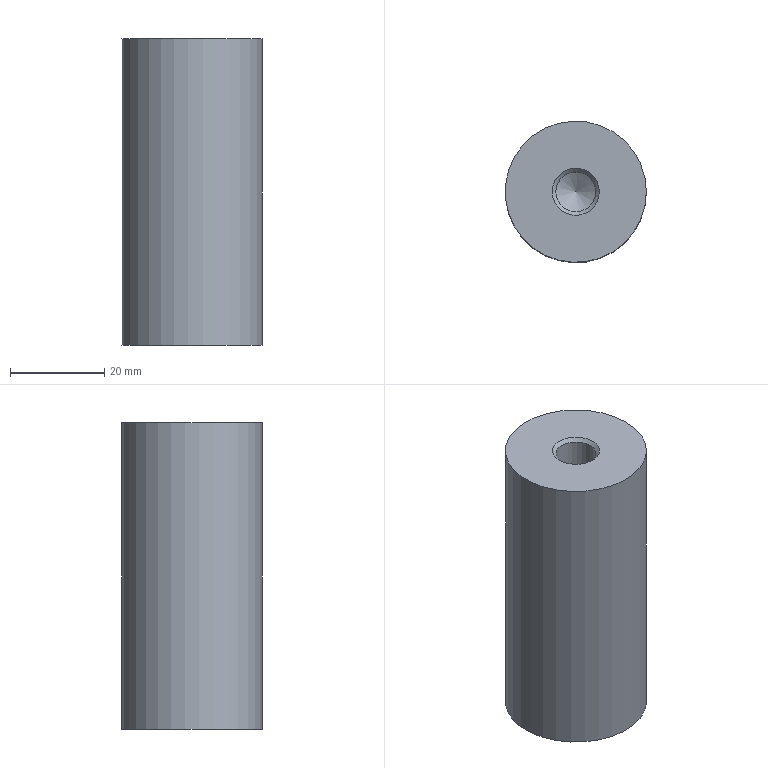Component | NX | SUPPORT_POST | 1 solid | 9 faces | box 30 x 30 x 65.25 mm | volume 42719 mm3 | cone 4 | cylinder 3 | plane 2 | commonest cylinder face diameters 8.5 x2 30 x1
STEP:
#1=CARTESIAN_POINT('',(0.,0.,0.));
#2=DIRECTION('',(0.,0.,1.));
#3=DIRECTION('',(1.,0.,0.));
#4=AXIS2_PLACEMENT_3D('',#1,#2,#3);
#5=CARTESIAN_POINT('',(16.898,274.878,173.246));
#6=VERTEX_POINT('',#5);
#7=CARTESIAN_POINT('',(1.898,274.878,173.246));
#8=DIRECTION('',(0.,0.,1.));
#9=DIRECTION('',(1.,0.,0.));
#10=AXIS2_PLACEMENT_3D('',#7,#8,#9);
#11=CIRCLE('',#10,15.);
#12=CARTESIAN_POINT('',(1.898,274.878,173.246));
#13=DIRECTION('',(0.,0.,-1.));
#14=DIRECTION('',(-1.,0.,0.));
#15=AXIS2_PLACEMENT_3D('',#12,#13,#14);
#16=CYLINDRICAL_SURFACE('',#15,15.);
#17=CARTESIAN_POINT('',(9.425,0.));
#18=DIRECTION('',(-1.,0.));
#19=VECTOR('',#18,1.);
#20=LINE('',#17,#19);
#21=(GEOMETRIC_REPRESENTATION_CONTEXT(2)PARAMETRIC_REPRESENTATION_CONTEXT()REPRESENTATION_CONTEXT('',''));
#22=DEFINITIONAL_REPRESENTATION('',(#20),#21);
#23=PCURVE('',#16,#22);
#24=CARTESIAN_POINT('',(1.898,274.878,173.246));
#25=DIRECTION('',(0.,0.,1.));
#26=DIRECTION('',(1.,0.,0.));
#27=AXIS2_PLACEMENT_3D('',#24,#25,#26);
#28=PLANE('',#27);
#29=CARTESIAN_POINT('',(0.,0.));
#30=DIRECTION('',(1.,0.));
#31=AXIS2_PLACEMENT_2D('',#29,#30);
#32=CIRCLE('',#31,15.);
#33=(GEOMETRIC_REPRESENTATION_CONTEXT(2)PARAMETRIC_REPRESENTATION_CONTEXT()REPRESENTATION_CONTEXT('',''));
#34=DEFINITIONAL_REPRESENTATION('',(#32),#33);
#35=PCURVE('',#28,#34);
#36=SURFACE_CURVE('',#11,(#23,#35),.PCURVE_S1.);
#37=EDGE_CURVE('',#6,#6,#36,.T.);
#38=ORIENTED_EDGE('',*,*,#37,.F.);
#39=CARTESIAN_POINT('',(16.898,274.878,107.996));
#40=VERTEX_POINT('',#39);
#41=CARTESIAN_POINT('',(16.898,274.878,173.246));
#42=CARTESIAN_POINT('',(16.898,274.878,107.996));
#43=B_SPLINE_CURVE_WITH_KNOTS('',1,(#41,#42),.UNSPECIFIED.,.F.,.F.,(2,2),(0.,65.25),.PIECEWISE_BEZIER_KNOTS.);
#44=CARTESIAN_POINT('',(9.425,0.));
#45=DIRECTION('',(0.,1.));
#46=VECTOR('',#45,1.);
#47=LINE('',#44,#46);
#48=(GEOMETRIC_REPRESENTATION_CONTEXT(2)PARAMETRIC_REPRESENTATION_CONTEXT()REPRESENTATION_CONTEXT('',''));
#49=DEFINITIONAL_REPRESENTATION('',(#47),#48);
#50=PCURVE('',#16,#49);
#51=CARTESIAN_POINT('',(3.142,0.));
#52=DIRECTION('',(0.,1.));
#53=VECTOR('',#52,1.);
#54=LINE('',#51,#53);
#55=(GEOMETRIC_REPRESENTATION_CONTEXT(2)PARAMETRIC_REPRESENTATION_CONTEXT()REPRESENTATION_CONTEXT('',''));
#56=DEFINITIONAL_REPRESENTATION('',(#54),#55);
#57=PCURVE('',#16,#56);
#58=SEAM_CURVE('',#43,(#50,#57),.PCURVE_S1.);
#59=EDGE_CURVE('',#6,#40,#58,.T.);
#60=ORIENTED_EDGE('',*,*,#59,.T.);
#61=CARTESIAN_POINT('',(1.898,274.878,107.996));
#62=DIRECTION('',(0.,0.,1.));
#63=DIRECTION('',(1.,0.,0.));
#64=AXIS2_PLACEMENT_3D('',#61,#62,#63);
#65=CIRCLE('',#64,15.);
#66=CARTESIAN_POINT('',(9.425,65.25));
#67=DIRECTION('',(-1.,0.));
#68=VECTOR('',#67,1.);
#69=LINE('',#66,#68);
#70=(GEOMETRIC_REPRESENTATION_CONTEXT(2)PARAMETRIC_REPRESENTATION_CONTEXT()REPRESENTATION_CONTEXT('',''));
#71=DEFINITIONAL_REPRESENTATION('',(#69),#70);
#72=PCURVE('',#16,#71);
#73=CARTESIAN_POINT('',(1.898,274.878,107.996));
#74=DIRECTION('',(0.,0.,1.));
#75=DIRECTION('',(1.,0.,0.));
#76=AXIS2_PLACEMENT_3D('',#73,#74,#75);
#77=PLANE('',#76);
#78=CARTESIAN_POINT('',(0.,0.));
#79=DIRECTION('',(1.,0.));
#80=AXIS2_PLACEMENT_2D('',#78,#79);
#81=CIRCLE('',#80,15.);
#82=(GEOMETRIC_REPRESENTATION_CONTEXT(2)PARAMETRIC_REPRESENTATION_CONTEXT()REPRESENTATION_CONTEXT('',''));
#83=DEFINITIONAL_REPRESENTATION('',(#81),#82);
#84=PCURVE('',#77,#83);
#85=SURFACE_CURVE('',#65,(#72,#84),.PCURVE_S1.);
#86=EDGE_CURVE('',#40,#40,#85,.T.);
#87=ORIENTED_EDGE('',*,*,#86,.T.);
#88=ORIENTED_EDGE('',*,*,#59,.F.);
#89=EDGE_LOOP('',(#38,#60,#87,#88));
#90=FACE_BOUND('',#89,.T.);
#91=ADVANCED_FACE('',(#90),#16,.T.);
#92=CARTESIAN_POINT('',(6.898,274.878,173.246));
#93=VERTEX_POINT('',#92);
#94=CARTESIAN_POINT('',(1.898,274.878,173.246));
#95=DIRECTION('',(0.,0.,1.));
#96=DIRECTION('',(1.,0.,0.));
#97=AXIS2_PLACEMENT_3D('',#94,#95,#96);
#98=CIRCLE('',#97,5.);
#99=CARTESIAN_POINT('',(0.,0.));
#100=DIRECTION('',(1.,0.));
#101=AXIS2_PLACEMENT_2D('',#99,#100);
#102=CIRCLE('',#101,5.);
#103=(GEOMETRIC_REPRESENTATION_CONTEXT(2)PARAMETRIC_REPRESENTATION_CONTEXT()REPRESENTATION_CONTEXT('',''));
#104=DEFINITIONAL_REPRESENTATION('',(#102),#103);
#105=PCURVE('',#28,#104);
#106=CARTESIAN_POINT('',(1.898,274.878,168.246));
#107=DIRECTION('',(0.,0.,1.));
#108=DIRECTION('',(1.,0.,0.));
#109=AXIS2_PLACEMENT_3D('',#106,#107,#108);
#110=CONICAL_SURFACE('',#109,0.,0.7854);
#111=CARTESIAN_POINT('',(0.,5.));
#112=DIRECTION('',(1.,0.));
#113=VECTOR('',#112,1.);
#114=LINE('',#111,#113);
#115=(GEOMETRIC_REPRESENTATION_CONTEXT(2)PARAMETRIC_REPRESENTATION_CONTEXT()REPRESENTATION_CONTEXT('',''));
#116=DEFINITIONAL_REPRESENTATION('',(#114),#115);
#117=PCURVE('',#110,#116);
#118=SURFACE_CURVE('',#98,(#105,#117),.PCURVE_S1.);
#119=EDGE_CURVE('',#93,#93,#118,.T.);
#120=ORIENTED_EDGE('',*,*,#119,.F.);
#121=EDGE_LOOP('',(#120));
#122=FACE_BOUND('',#121,.T.);
#123=ORIENTED_EDGE('',*,*,#37,.T.);
#124=EDGE_LOOP('',(#123));
#125=FACE_BOUND('',#124,.T.);
#126=ADVANCED_FACE('',(#122,#125),#28,.T.);
#127=CARTESIAN_POINT('',(6.898,274.878,107.996));
#128=VERTEX_POINT('',#127);
#129=CARTESIAN_POINT('',(-3.102,274.878,107.996));
#130=VERTEX_POINT('',#129);
#131=CARTESIAN_POINT('',(1.898,274.878,107.996));
#132=DIRECTION('',(0.,0.,1.));
#133=DIRECTION('',(1.,0.,0.));
#134=AXIS2_PLACEMENT_3D('',#131,#132,#133);
#135=CIRCLE('',#134,5.);
#136=CARTESIAN_POINT('',(0.,0.));
#137=DIRECTION('',(1.,0.));
#138=AXIS2_PLACEMENT_2D('',#136,#137);
#139=CIRCLE('',#138,5.);
#140=(GEOMETRIC_REPRESENTATION_CONTEXT(2)PARAMETRIC_REPRESENTATION_CONTEXT()REPRESENTATION_CONTEXT('',''));
#141=DEFINITIONAL_REPRESENTATION('',(#139),#140);
#142=PCURVE('',#77,#141);
#143=CARTESIAN_POINT('',(1.898,274.878,112.996));
#144=DIRECTION('',(0.,0.,-1.));
#145=DIRECTION('',(-1.,0.,0.));
#146=AXIS2_PLACEMENT_3D('',#143,#144,#145);
#147=CONICAL_SURFACE('',#146,0.,0.7854);
#148=CARTESIAN_POINT('',(3.142,5.));
#149=DIRECTION('',(-1.,0.));
#150=VECTOR('',#149,1.);
#151=LINE('',#148,#150);
#152=(GEOMETRIC_REPRESENTATION_CONTEXT(2)PARAMETRIC_REPRESENTATION_CONTEXT()REPRESENTATION_CONTEXT('',''));
#153=DEFINITIONAL_REPRESENTATION('',(#151),#152);
#154=PCURVE('',#147,#153);
#155=SURFACE_CURVE('',#135,(#142,#154),.PCURVE_S1.);
#156=EDGE_CURVE('',#128,#130,#155,.T.);
#157=ORIENTED_EDGE('',*,*,#156,.T.);
#158=CARTESIAN_POINT('',(1.898,274.878,107.996));
#159=DIRECTION('',(0.,0.,1.));
#160=DIRECTION('',(1.,0.,0.));
#161=AXIS2_PLACEMENT_3D('',#158,#159,#160);
#162=CIRCLE('',#161,5.);
#163=CARTESIAN_POINT('',(0.,0.));
#164=DIRECTION('',(1.,0.));
#165=AXIS2_PLACEMENT_2D('',#163,#164);
#166=CIRCLE('',#165,5.);
#167=(GEOMETRIC_REPRESENTATION_CONTEXT(2)PARAMETRIC_REPRESENTATION_CONTEXT()REPRESENTATION_CONTEXT('',''));
#168=DEFINITIONAL_REPRESENTATION('',(#166),#167);
#169=PCURVE('',#77,#168);
#170=CARTESIAN_POINT('',(9.425,5.));
#171=DIRECTION('',(-1.,0.));
#172=VECTOR('',#171,1.);
#173=LINE('',#170,#172);
#174=(GEOMETRIC_REPRESENTATION_CONTEXT(2)PARAMETRIC_REPRESENTATION_CONTEXT()REPRESENTATION_CONTEXT('',''));
#175=DEFINITIONAL_REPRESENTATION('',(#173),#174);
#176=PCURVE('',#147,#175);
#177=SURFACE_CURVE('',#162,(#169,#176),.PCURVE_S1.);
#178=EDGE_CURVE('',#130,#128,#177,.T.);
#179=ORIENTED_EDGE('',*,*,#178,.T.);
#180=EDGE_LOOP('',(#157,#179));
#181=FACE_BOUND('',#180,.T.);
#182=ORIENTED_EDGE('',*,*,#86,.F.);
#183=EDGE_LOOP('',(#182));
#184=FACE_BOUND('',#183,.T.);
#185=ADVANCED_FACE('',(#181,#184),#77,.F.);
#186=ORIENTED_EDGE('',*,*,#119,.F.);
#187=CARTESIAN_POINT('',(6.148,274.878,172.496));
#188=VERTEX_POINT('',#187);
#189=CARTESIAN_POINT('',(6.148,274.878,172.496));
#190=CARTESIAN_POINT('',(6.898,274.878,173.246));
#191=B_SPLINE_CURVE_WITH_KNOTS('',1,(#189,#190),.UNSPECIFIED.,.F.,.F.,(2,2),(6.01,7.071),.PIECEWISE_BEZIER_KNOTS.);
#192=CARTESIAN_POINT('',(0.,0.));
#193=DIRECTION('',(0.,1.));
#194=VECTOR('',#193,1.);
#195=LINE('',#192,#194);
#196=(GEOMETRIC_REPRESENTATION_CONTEXT(2)PARAMETRIC_REPRESENTATION_CONTEXT()REPRESENTATION_CONTEXT('',''));
#197=DEFINITIONAL_REPRESENTATION('',(#195),#196);
#198=PCURVE('',#110,#197);
#199=CARTESIAN_POINT('',(6.283,0.));
#200=DIRECTION('',(0.,1.));
#201=VECTOR('',#200,1.);
#202=LINE('',#199,#201);
#203=(GEOMETRIC_REPRESENTATION_CONTEXT(2)PARAMETRIC_REPRESENTATION_CONTEXT()REPRESENTATION_CONTEXT('',''));
#204=DEFINITIONAL_REPRESENTATION('',(#202),#203);
#205=PCURVE('',#110,#204);
#206=SEAM_CURVE('',#191,(#198,#205),.PCURVE_S1.);
#207=EDGE_CURVE('',#188,#93,#206,.T.);
#208=ORIENTED_EDGE('',*,*,#207,.F.);
#209=CARTESIAN_POINT('',(1.898,274.878,172.496));
#210=DIRECTION('',(0.,0.,1.));
#211=DIRECTION('',(1.,0.,0.));
#212=AXIS2_PLACEMENT_3D('',#209,#210,#211);
#213=CIRCLE('',#212,4.25);
#214=CARTESIAN_POINT('',(0.,4.25));
#215=DIRECTION('',(1.,0.));
#216=VECTOR('',#215,1.);
#217=LINE('',#214,#216);
#218=(GEOMETRIC_REPRESENTATION_CONTEXT(2)PARAMETRIC_REPRESENTATION_CONTEXT()REPRESENTATION_CONTEXT('',''));
#219=DEFINITIONAL_REPRESENTATION('',(#217),#218);
#220=PCURVE('',#110,#219);
#221=CARTESIAN_POINT('',(1.898,274.878,173.246));
#222=DIRECTION('',(0.,0.,-1.));
#223=DIRECTION('',(-1.,0.,0.));
#224=AXIS2_PLACEMENT_3D('',#221,#222,#223);
#225=CYLINDRICAL_SURFACE('',#224,4.25);
#226=CARTESIAN_POINT('',(9.425,0.75));
#227=DIRECTION('',(-1.,0.));
#228=VECTOR('',#227,1.);
#229=LINE('',#226,#228);
#230=(GEOMETRIC_REPRESENTATION_CONTEXT(2)PARAMETRIC_REPRESENTATION_CONTEXT()REPRESENTATION_CONTEXT('',''));
#231=DEFINITIONAL_REPRESENTATION('',(#229),#230);
#232=PCURVE('',#225,#231);
#233=SURFACE_CURVE('',#213,(#220,#232),.PCURVE_S1.);
#234=EDGE_CURVE('',#188,#188,#233,.T.);
#235=ORIENTED_EDGE('',*,*,#234,.T.);
#236=ORIENTED_EDGE('',*,*,#207,.T.);
#237=EDGE_LOOP('',(#186,#208,#235,#236));
#238=FACE_BOUND('',#237,.F.);
#239=ADVANCED_FACE('',(#238),#110,.F.);
#240=CARTESIAN_POINT('',(6.148,274.878,145.746));
#241=VERTEX_POINT('',#240);
#242=CARTESIAN_POINT('',(-2.352,274.878,145.746));
#243=VERTEX_POINT('',#242);
#244=CARTESIAN_POINT('',(1.898,274.878,145.746));
#245=DIRECTION('',(0.,0.,1.));
#246=DIRECTION('',(-1.,0.,0.));
#247=AXIS2_PLACEMENT_3D('',#244,#245,#246);
#248=CIRCLE('',#247,4.25);
#249=CARTESIAN_POINT('',(1.898,274.878,145.746));
#250=DIRECTION('',(0.,0.,1.));
#251=DIRECTION('',(1.,0.,0.));
#252=AXIS2_PLACEMENT_3D('',#249,#250,#251);
#253=CONICAL_SURFACE('',#252,4.25,1.03);
#254=CARTESIAN_POINT('',(-3.142,0.));
#255=DIRECTION('',(1.,0.));
#256=VECTOR('',#255,1.);
#257=LINE('',#254,#256);
#258=(GEOMETRIC_REPRESENTATION_CONTEXT(2)PARAMETRIC_REPRESENTATION_CONTEXT()REPRESENTATION_CONTEXT('',''));
#259=DEFINITIONAL_REPRESENTATION('',(#257),#258);
#260=PCURVE('',#253,#259);
#261=CARTESIAN_POINT('',(12.566,27.5));
#262=DIRECTION('',(-1.,0.));
#263=VECTOR('',#262,1.);
#264=LINE('',#261,#263);
#265=(GEOMETRIC_REPRESENTATION_CONTEXT(2)PARAMETRIC_REPRESENTATION_CONTEXT()REPRESENTATION_CONTEXT('',''));
#266=DEFINITIONAL_REPRESENTATION('',(#264),#265);
#267=PCURVE('',#225,#266);
#268=SURFACE_CURVE('',#248,(#260,#267),.PCURVE_S1.);
#269=EDGE_CURVE('',#241,#243,#268,.T.);
#270=ORIENTED_EDGE('',*,*,#269,.F.);
#271=CARTESIAN_POINT('',(1.898,274.878,143.193));
#272=VERTEX_POINT('',#271);
#273=CARTESIAN_POINT('',(1.898,274.878,143.193));
#274=CARTESIAN_POINT('',(6.148,274.878,145.746));
#275=B_SPLINE_CURVE_WITH_KNOTS('',1,(#273,#274),.UNSPECIFIED.,.F.,.F.,(2,2),(-4.958,0.),.PIECEWISE_BEZIER_KNOTS.);
#276=CARTESIAN_POINT('',(0.,0.));
#277=DIRECTION('',(0.,1.));
#278=VECTOR('',#277,1.);
#279=LINE('',#276,#278);
#280=(GEOMETRIC_REPRESENTATION_CONTEXT(2)PARAMETRIC_REPRESENTATION_CONTEXT()REPRESENTATION_CONTEXT('',''));
#281=DEFINITIONAL_REPRESENTATION('',(#279),#280);
#282=PCURVE('',#253,#281);
#283=CARTESIAN_POINT('',(6.283,0.));
#284=DIRECTION('',(0.,1.));
#285=VECTOR('',#284,1.);
#286=LINE('',#283,#285);
#287=(GEOMETRIC_REPRESENTATION_CONTEXT(2)PARAMETRIC_REPRESENTATION_CONTEXT()REPRESENTATION_CONTEXT('',''));
#288=DEFINITIONAL_REPRESENTATION('',(#286),#287);
#289=PCURVE('',#253,#288);
#290=SEAM_CURVE('',#275,(#282,#289),.PCURVE_S1.);
#291=EDGE_CURVE('',#272,#241,#290,.T.);
#292=ORIENTED_EDGE('',*,*,#291,.F.);
#293=ORIENTED_EDGE('',*,*,#291,.T.);
#294=CARTESIAN_POINT('',(1.898,274.878,145.746));
#295=DIRECTION('',(0.,0.,1.));
#296=DIRECTION('',(-1.,0.,0.));
#297=AXIS2_PLACEMENT_3D('',#294,#295,#296);
#298=CIRCLE('',#297,4.25);
#299=CARTESIAN_POINT('',(3.142,0.));
#300=DIRECTION('',(1.,0.));
#301=VECTOR('',#300,1.);
#302=LINE('',#299,#301);
#303=(GEOMETRIC_REPRESENTATION_CONTEXT(2)PARAMETRIC_REPRESENTATION_CONTEXT()REPRESENTATION_CONTEXT('',''));
#304=DEFINITIONAL_REPRESENTATION('',(#302),#303);
#305=PCURVE('',#253,#304);
#306=CARTESIAN_POINT('',(6.283,27.5));
#307=DIRECTION('',(-1.,0.));
#308=VECTOR('',#307,1.);
#309=LINE('',#306,#308);
#310=(GEOMETRIC_REPRESENTATION_CONTEXT(2)PARAMETRIC_REPRESENTATION_CONTEXT()REPRESENTATION_CONTEXT('',''));
#311=DEFINITIONAL_REPRESENTATION('',(#309),#310);
#312=PCURVE('',#225,#311);
#313=SURFACE_CURVE('',#298,(#305,#312),.PCURVE_S1.);
#314=EDGE_CURVE('',#243,#241,#313,.T.);
#315=ORIENTED_EDGE('',*,*,#314,.F.);
#316=EDGE_LOOP('',(#270,#292,#293,#315));
#317=FACE_BOUND('',#316,.F.);
#318=ADVANCED_FACE('',(#317),#253,.F.);
#319=ORIENTED_EDGE('',*,*,#234,.F.);
#320=CARTESIAN_POINT('',(6.148,274.878,172.496));
#321=CARTESIAN_POINT('',(6.148,274.878,145.746));
#322=B_SPLINE_CURVE_WITH_KNOTS('',1,(#320,#321),.UNSPECIFIED.,.F.,.F.,(2,2),(0.75,27.5),.PIECEWISE_BEZIER_KNOTS.);
#323=CARTESIAN_POINT('',(9.425,0.));
#324=DIRECTION('',(0.,1.));
#325=VECTOR('',#324,1.);
#326=LINE('',#323,#325);
#327=(GEOMETRIC_REPRESENTATION_CONTEXT(2)PARAMETRIC_REPRESENTATION_CONTEXT()REPRESENTATION_CONTEXT('',''));
#328=DEFINITIONAL_REPRESENTATION('',(#326),#327);
#329=PCURVE('',#225,#328);
#330=CARTESIAN_POINT('',(3.142,0.));
#331=DIRECTION('',(0.,1.));
#332=VECTOR('',#331,1.);
#333=LINE('',#330,#332);
#334=(GEOMETRIC_REPRESENTATION_CONTEXT(2)PARAMETRIC_REPRESENTATION_CONTEXT()REPRESENTATION_CONTEXT('',''));
#335=DEFINITIONAL_REPRESENTATION('',(#333),#334);
#336=PCURVE('',#225,#335);
#337=SEAM_CURVE('',#322,(#329,#336),.PCURVE_S1.);
#338=EDGE_CURVE('',#188,#241,#337,.T.);
#339=ORIENTED_EDGE('',*,*,#338,.T.);
#340=ORIENTED_EDGE('',*,*,#269,.T.);
#341=ORIENTED_EDGE('',*,*,#314,.T.);
#342=ORIENTED_EDGE('',*,*,#338,.F.);
#343=EDGE_LOOP('',(#319,#339,#340,#341,#342));
#344=FACE_BOUND('',#343,.F.);
#345=ADVANCED_FACE('',(#344),#225,.F.);
#346=CARTESIAN_POINT('',(-2.352,274.878,108.746));
#347=VERTEX_POINT('',#346);
#348=CARTESIAN_POINT('',(1.898,274.878,108.746));
#349=DIRECTION('',(0.,0.,-1.));
#350=DIRECTION('',(-1.,0.,0.));
#351=AXIS2_PLACEMENT_3D('',#348,#349,#350);
#352=CIRCLE('',#351,4.25);
#353=CARTESIAN_POINT('',(0.,4.25));
#354=DIRECTION('',(1.,0.));
#355=VECTOR('',#354,1.);
#356=LINE('',#353,#355);
#357=(GEOMETRIC_REPRESENTATION_CONTEXT(2)PARAMETRIC_REPRESENTATION_CONTEXT()REPRESENTATION_CONTEXT('',''));
#358=DEFINITIONAL_REPRESENTATION('',(#356),#357);
#359=PCURVE('',#147,#358);
#360=CARTESIAN_POINT('',(1.898,274.878,107.996));
#361=DIRECTION('',(0.,0.,1.));
#362=DIRECTION('',(1.,0.,0.));
#363=AXIS2_PLACEMENT_3D('',#360,#361,#362);
#364=CYLINDRICAL_SURFACE('',#363,4.25);
#365=CARTESIAN_POINT('',(9.425,0.75));
#366=DIRECTION('',(-1.,0.));
#367=VECTOR('',#366,1.);
#368=LINE('',#365,#367);
#369=(GEOMETRIC_REPRESENTATION_CONTEXT(2)PARAMETRIC_REPRESENTATION_CONTEXT()REPRESENTATION_CONTEXT('',''));
#370=DEFINITIONAL_REPRESENTATION('',(#368),#369);
#371=PCURVE('',#364,#370);
#372=SURFACE_CURVE('',#352,(#359,#371),.PCURVE_S1.);
#373=EDGE_CURVE('',#347,#347,#372,.T.);
#374=ORIENTED_EDGE('',*,*,#373,.T.);
#375=CARTESIAN_POINT('',(-2.352,274.878,108.746));
#376=CARTESIAN_POINT('',(-3.102,274.878,107.996));
#377=B_SPLINE_CURVE_WITH_KNOTS('',1,(#375,#376),.UNSPECIFIED.,.F.,.F.,(2,2),(6.01,7.071),.PIECEWISE_BEZIER_KNOTS.);
#378=CARTESIAN_POINT('',(6.283,0.));
#379=DIRECTION('',(0.,1.));
#380=VECTOR('',#379,1.);
#381=LINE('',#378,#380);
#382=(GEOMETRIC_REPRESENTATION_CONTEXT(2)PARAMETRIC_REPRESENTATION_CONTEXT()REPRESENTATION_CONTEXT('',''));
#383=DEFINITIONAL_REPRESENTATION('',(#381),#382);
#384=PCURVE('',#147,#383);
#385=CARTESIAN_POINT('',(0.,0.));
#386=DIRECTION('',(0.,1.));
#387=VECTOR('',#386,1.);
#388=LINE('',#385,#387);
#389=(GEOMETRIC_REPRESENTATION_CONTEXT(2)PARAMETRIC_REPRESENTATION_CONTEXT()REPRESENTATION_CONTEXT('',''));
#390=DEFINITIONAL_REPRESENTATION('',(#388),#389);
#391=PCURVE('',#147,#390);
#392=SEAM_CURVE('',#377,(#384,#391),.PCURVE_S1.);
#393=EDGE_CURVE('',#347,#130,#392,.T.);
#394=ORIENTED_EDGE('',*,*,#393,.T.);
#395=ORIENTED_EDGE('',*,*,#178,.T.);
#396=ORIENTED_EDGE('',*,*,#156,.T.);
#397=ORIENTED_EDGE('',*,*,#393,.F.);
#398=EDGE_LOOP('',(#374,#394,#395,#396,#397));
#399=FACE_BOUND('',#398,.F.);
#400=ADVANCED_FACE('',(#399),#147,.F.);
#401=CARTESIAN_POINT('',(-2.352,274.878,138.496));
#402=VERTEX_POINT('',#401);
#403=CARTESIAN_POINT('',(6.148,274.878,138.496));
#404=VERTEX_POINT('',#403);
#405=CARTESIAN_POINT('',(1.898,274.878,138.496));
#406=DIRECTION('',(0.,0.,-1.));
#407=DIRECTION('',(1.,0.,0.));
#408=AXIS2_PLACEMENT_3D('',#405,#406,#407);
#409=CIRCLE('',#408,4.25);
#410=CARTESIAN_POINT('',(1.898,274.878,138.496));
#411=DIRECTION('',(0.,0.,-1.));
#412=DIRECTION('',(-1.,0.,0.));
#413=AXIS2_PLACEMENT_3D('',#410,#411,#412);
#414=CONICAL_SURFACE('',#413,4.25,1.03);
#415=CARTESIAN_POINT('',(-3.142,0.));
#416=DIRECTION('',(1.,0.));
#417=VECTOR('',#416,1.);
#418=LINE('',#415,#417);
#419=(GEOMETRIC_REPRESENTATION_CONTEXT(2)PARAMETRIC_REPRESENTATION_CONTEXT()REPRESENTATION_CONTEXT('',''));
#420=DEFINITIONAL_REPRESENTATION('',(#418),#419);
#421=PCURVE('',#414,#420);
#422=CARTESIAN_POINT('',(12.566,30.5));
#423=DIRECTION('',(-1.,0.));
#424=VECTOR('',#423,1.);
#425=LINE('',#422,#424);
#426=(GEOMETRIC_REPRESENTATION_CONTEXT(2)PARAMETRIC_REPRESENTATION_CONTEXT()REPRESENTATION_CONTEXT('',''));
#427=DEFINITIONAL_REPRESENTATION('',(#425),#426);
#428=PCURVE('',#364,#427);
#429=SURFACE_CURVE('',#409,(#421,#428),.PCURVE_S1.);
#430=EDGE_CURVE('',#402,#404,#429,.T.);
#431=ORIENTED_EDGE('',*,*,#430,.F.);
#432=CARTESIAN_POINT('',(1.898,274.878,141.05));
#433=VERTEX_POINT('',#432);
#434=CARTESIAN_POINT('',(1.898,274.878,141.05));
#435=CARTESIAN_POINT('',(-2.352,274.878,138.496));
#436=B_SPLINE_CURVE_WITH_KNOTS('',1,(#434,#435),.UNSPECIFIED.,.F.,.F.,(2,2),(-4.958,0.),.PIECEWISE_BEZIER_KNOTS.);
#437=CARTESIAN_POINT('',(0.,0.));
#438=DIRECTION('',(0.,1.));
#439=VECTOR('',#438,1.);
#440=LINE('',#437,#439);
#441=(GEOMETRIC_REPRESENTATION_CONTEXT(2)PARAMETRIC_REPRESENTATION_CONTEXT()REPRESENTATION_CONTEXT('',''));
#442=DEFINITIONAL_REPRESENTATION('',(#440),#441);
#443=PCURVE('',#414,#442);
#444=CARTESIAN_POINT('',(6.283,0.));
#445=DIRECTION('',(0.,1.));
#446=VECTOR('',#445,1.);
#447=LINE('',#444,#446);
#448=(GEOMETRIC_REPRESENTATION_CONTEXT(2)PARAMETRIC_REPRESENTATION_CONTEXT()REPRESENTATION_CONTEXT('',''));
#449=DEFINITIONAL_REPRESENTATION('',(#447),#448);
#450=PCURVE('',#414,#449);
#451=SEAM_CURVE('',#436,(#443,#450),.PCURVE_S1.);
#452=EDGE_CURVE('',#433,#402,#451,.T.);
#453=ORIENTED_EDGE('',*,*,#452,.F.);
#454=ORIENTED_EDGE('',*,*,#452,.T.);
#455=CARTESIAN_POINT('',(1.898,274.878,138.496));
#456=DIRECTION('',(0.,0.,-1.));
#457=DIRECTION('',(1.,0.,0.));
#458=AXIS2_PLACEMENT_3D('',#455,#456,#457);
#459=CIRCLE('',#458,4.25);
#460=CARTESIAN_POINT('',(3.142,0.));
#461=DIRECTION('',(1.,0.));
#462=VECTOR('',#461,1.);
#463=LINE('',#460,#462);
#464=(GEOMETRIC_REPRESENTATION_CONTEXT(2)PARAMETRIC_REPRESENTATION_CONTEXT()REPRESENTATION_CONTEXT('',''));
#465=DEFINITIONAL_REPRESENTATION('',(#463),#464);
#466=PCURVE('',#414,#465);
#467=CARTESIAN_POINT('',(6.283,30.5));
#468=DIRECTION('',(-1.,0.));
#469=VECTOR('',#468,1.);
#470=LINE('',#467,#469);
#471=(GEOMETRIC_REPRESENTATION_CONTEXT(2)PARAMETRIC_REPRESENTATION_CONTEXT()REPRESENTATION_CONTEXT('',''));
#472=DEFINITIONAL_REPRESENTATION('',(#470),#471);
#473=PCURVE('',#364,#472);
#474=SURFACE_CURVE('',#459,(#466,#473),.PCURVE_S1.);
#475=EDGE_CURVE('',#404,#402,#474,.T.);
#476=ORIENTED_EDGE('',*,*,#475,.F.);
#477=EDGE_LOOP('',(#431,#453,#454,#476));
#478=FACE_BOUND('',#477,.F.);
#479=ADVANCED_FACE('',(#478),#414,.F.);
#480=ORIENTED_EDGE('',*,*,#373,.F.);
#481=CARTESIAN_POINT('',(-2.352,274.878,108.746));
#482=CARTESIAN_POINT('',(-2.352,274.878,138.496));
#483=B_SPLINE_CURVE_WITH_KNOTS('',1,(#481,#482),.UNSPECIFIED.,.F.,.F.,(2,2),(0.75,30.5),.PIECEWISE_BEZIER_KNOTS.);
#484=CARTESIAN_POINT('',(9.425,0.));
#485=DIRECTION('',(0.,1.));
#486=VECTOR('',#485,1.);
#487=LINE('',#484,#486);
#488=(GEOMETRIC_REPRESENTATION_CONTEXT(2)PARAMETRIC_REPRESENTATION_CONTEXT()REPRESENTATION_CONTEXT('',''));
#489=DEFINITIONAL_REPRESENTATION('',(#487),#488);
#490=PCURVE('',#364,#489);
#491=CARTESIAN_POINT('',(3.142,0.));
#492=DIRECTION('',(0.,1.));
#493=VECTOR('',#492,1.);
#494=LINE('',#491,#493);
#495=(GEOMETRIC_REPRESENTATION_CONTEXT(2)PARAMETRIC_REPRESENTATION_CONTEXT()REPRESENTATION_CONTEXT('',''));
#496=DEFINITIONAL_REPRESENTATION('',(#494),#495);
#497=PCURVE('',#364,#496);
#498=SEAM_CURVE('',#483,(#490,#497),.PCURVE_S1.);
#499=EDGE_CURVE('',#347,#402,#498,.T.);
#500=ORIENTED_EDGE('',*,*,#499,.T.);
#501=ORIENTED_EDGE('',*,*,#430,.T.);
#502=ORIENTED_EDGE('',*,*,#475,.T.);
#503=ORIENTED_EDGE('',*,*,#499,.F.);
#504=EDGE_LOOP('',(#480,#500,#501,#502,#503));
#505=FACE_BOUND('',#504,.F.);
#506=ADVANCED_FACE('',(#505),#364,.F.);
#507=CLOSED_SHELL('',(#91,#126,#185,#239,#318,#345,#400,#479,#506));
#508=MANIFOLD_SOLID_BREP('',#507);
#509=(LENGTH_UNIT()NAMED_UNIT(*)SI_UNIT(.MILLI.,.METRE.));
#510=UNCERTAINTY_MEASURE_WITH_UNIT(LENGTH_MEASURE(0.000005),#509,'','');
#511=(NAMED_UNIT(*)PLANE_ANGLE_UNIT()SI_UNIT($,.RADIAN.));
#512=(NAMED_UNIT(*)SI_UNIT($,.STERADIAN.)SOLID_ANGLE_UNIT());
#513=(GEOMETRIC_REPRESENTATION_CONTEXT(3)GLOBAL_UNCERTAINTY_ASSIGNED_CONTEXT((#510))GLOBAL_UNIT_ASSIGNED_CONTEXT((#509,#511,#512))REPRESENTATION_CONTEXT('',''));
#514=ADVANCED_BREP_SHAPE_REPRESENTATION('',(#4,#508),#513);